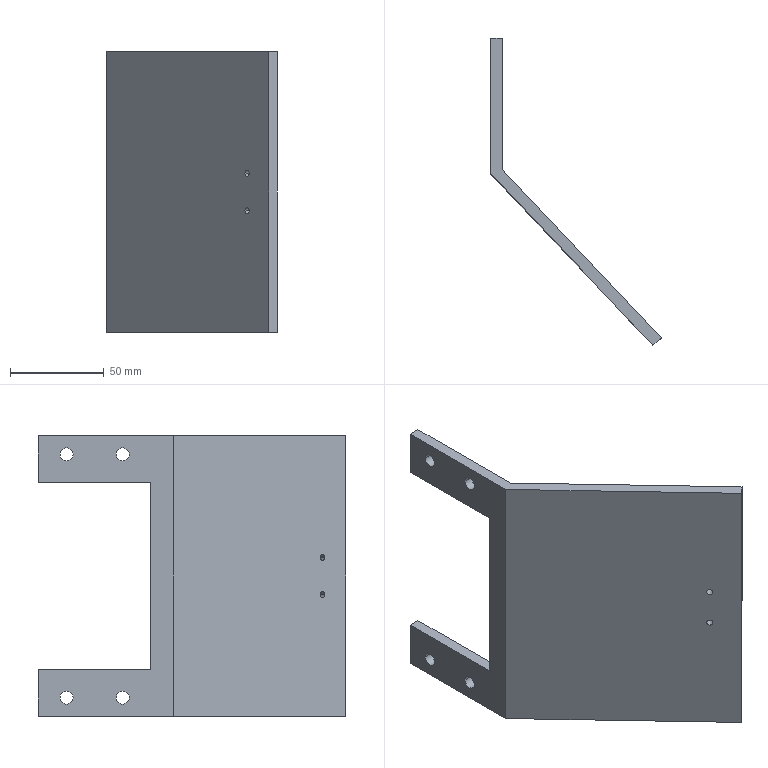Component | SolidWorks | ClampingMechanism-1_SupportPlate-1 | 1 solid | 24 faces | box 91 x 164.12 x 150 mm | volume 139535 mm3 | cylinder 12 | plane 12 | commonest cylinder face diameters 7 x8 3.3 x4
build123d program:
from build123d import *

# Parameters (mm, degrees)
BOSS_EXTRUDE1_DEPTH   = 75
SKETCH2_R             = 3.5
SKETCH2_W             = 120
SKETCH2_H             = 100
CUT_EXTRUDE1_DEPTH    = 10
M4_TAPPED_HOLE1_D     = 3.3
M4_TAPPED_HOLE1_DEPTH = 10.1
M4_TAPPED_HOLE1_TIP   = 0.9914


with BuildPart() as part:
    # Sketch1 → Boss-Extrude1 (new, symmetric)
    with BuildSketch(Plane.XY):
        Polygon((0, 0), (90, 85), (160, 85), (160, 91), (87.615, 91), (-4.12, 4.362), align=None)
    extrude(amount=BOSS_EXTRUDE1_DEPTH, both=True)

    # Sketch2 → Cut-Extrude1 (cut)
    with BuildSketch(Plane(origin=(0, 91, 0), x_dir=(1, 0, 0), z_dir=(0, 1, 0))):
        with Locations(Location((115, 65, 0), (0, 0, 180))):
            Circle(SKETCH2_R)
        with Locations(Location((145, 65, 0), (0, 0, 180))):
            Circle(SKETCH2_R)
        with Locations(Location((145, -65, 0), (0, 0, 180))):
            Circle(SKETCH2_R)
        with Locations(Location((115, -65, 0), (0, 0, 180))):
            Circle(SKETCH2_R)
        with Locations((160, 0)):
            Rectangle(SKETCH2_W, SKETCH2_H)
    extrude(amount=-CUT_EXTRUDE1_DEPTH, mode=Mode.SUBTRACT)

    # M4 Tapped Hole1
    with Locations(Plane(origin=(-4.12, 4.362, 0), x_dir=(0.727, 0.6866, 0), z_dir=(-0.6866, 0.727, 0))):
        with Locations((17, 10), (17, -10)):
            Hole(M4_TAPPED_HOLE1_D / 2, depth=M4_TAPPED_HOLE1_DEPTH)
            with Locations((0, 0, -(M4_TAPPED_HOLE1_DEPTH + M4_TAPPED_HOLE1_TIP / 2))):  # 118° drill point
                Cone(0, M4_TAPPED_HOLE1_D / 2, M4_TAPPED_HOLE1_TIP, mode=Mode.SUBTRACT)


solid = part.part

# Placed as in the assembly
solid = solid.moved(Location((-235, -250, -542.97), (0, 0, 90)))
STEP:
#1=COLOUR_RGB('',0.7922,0.8196,0.9333);
#2=FILL_AREA_STYLE_COLOUR('',#1);
#3=FILL_AREA_STYLE('',(#2));
#4=SURFACE_STYLE_FILL_AREA(#3);
#5=SURFACE_SIDE_STYLE('',(#4));
#6=SURFACE_STYLE_USAGE(.BOTH.,#5);
#7=PRESENTATION_STYLE_ASSIGNMENT((#6));
#8=CARTESIAN_POINT('',(-9.756,-9.309,-21.77));
#9=VERTEX_POINT('',#8);
#10=CARTESIAN_POINT('',(-9.667,-9.403,-21.77));
#11=VERTEX_POINT('',#10);
#12=CARTESIAN_POINT('',(-9.712,-9.356,-21.77));
#13=DIRECTION('',(-0.727,-0.6866,0.));
#14=DIRECTION('',(0.6866,-0.727,0.));
#15=AXIS2_PLACEMENT_3D('',#12,#13,#14);
#16=CIRCLE('',#15,0.06496);
#17=EDGE_CURVE('',#9,#11,#16,.T.);
#18=ORIENTED_EDGE('',*,*,#17,.F.);
#19=CARTESIAN_POINT('',(-9.928,-9.471,-21.77));
#20=VERTEX_POINT('',#19);
#21=CARTESIAN_POINT('',(-9.928,-9.471,-21.77));
#22=DIRECTION('',(-0.727,-0.6866,0.));
#23=VECTOR('',#22,39.37);
#24=LINE('',#21,#23);
#25=EDGE_CURVE('',#9,#20,#24,.T.);
#26=ORIENTED_EDGE('',*,*,#25,.T.);
#27=CARTESIAN_POINT('',(-9.839,-9.565,-21.77));
#28=VERTEX_POINT('',#27);
#29=CARTESIAN_POINT('',(-9.883,-9.518,-21.77));
#30=DIRECTION('',(-0.727,-0.6866,0.));
#31=DIRECTION('',(0.6866,-0.727,0.));
#32=AXIS2_PLACEMENT_3D('',#29,#30,#31);
#33=CIRCLE('',#32,0.06496);
#34=EDGE_CURVE('',#20,#28,#33,.T.);
#35=ORIENTED_EDGE('',*,*,#34,.T.);
#36=CARTESIAN_POINT('',(-9.839,-9.565,-21.77));
#37=DIRECTION('',(-0.727,-0.6866,0.));
#38=VECTOR('',#37,39.37);
#39=LINE('',#36,#38);
#40=EDGE_CURVE('',#11,#28,#39,.T.);
#41=ORIENTED_EDGE('',*,*,#40,.F.);
#42=EDGE_LOOP('',(#18,#26,#35,#41));
#43=FACE_OUTER_BOUND('',#42,.T.);
#44=CARTESIAN_POINT('',(-9.883,-9.518,-21.77));
#45=DIRECTION('',(-0.727,-0.6866,0.));
#46=DIRECTION('',(0.6866,-0.727,0.));
#47=AXIS2_PLACEMENT_3D('',#44,#45,#46);
#48=CYLINDRICAL_SURFACE('',#47,0.06496);
#49=ADVANCED_FACE('',(#43),#48,.F.);
#50=CARTESIAN_POINT('',(-9.756,-9.309,-20.983));
#51=VERTEX_POINT('',#50);
#52=CARTESIAN_POINT('',(-9.667,-9.403,-20.983));
#53=VERTEX_POINT('',#52);
#54=CARTESIAN_POINT('',(-9.712,-9.356,-20.983));
#55=DIRECTION('',(-0.727,-0.6866,0.));
#56=DIRECTION('',(0.6866,-0.727,0.));
#57=AXIS2_PLACEMENT_3D('',#54,#55,#56);
#58=CIRCLE('',#57,0.06496);
#59=EDGE_CURVE('',#51,#53,#58,.T.);
#60=ORIENTED_EDGE('',*,*,#59,.F.);
#61=CARTESIAN_POINT('',(-9.928,-9.471,-20.983));
#62=VERTEX_POINT('',#61);
#63=CARTESIAN_POINT('',(-9.928,-9.471,-20.983));
#64=DIRECTION('',(-0.727,-0.6866,0.));
#65=VECTOR('',#64,39.37);
#66=LINE('',#63,#65);
#67=EDGE_CURVE('',#51,#62,#66,.T.);
#68=ORIENTED_EDGE('',*,*,#67,.T.);
#69=CARTESIAN_POINT('',(-9.839,-9.565,-20.983));
#70=VERTEX_POINT('',#69);
#71=CARTESIAN_POINT('',(-9.883,-9.518,-20.983));
#72=DIRECTION('',(-0.727,-0.6866,0.));
#73=DIRECTION('',(0.6866,-0.727,0.));
#74=AXIS2_PLACEMENT_3D('',#71,#72,#73);
#75=CIRCLE('',#74,0.06496);
#76=EDGE_CURVE('',#62,#70,#75,.T.);
#77=ORIENTED_EDGE('',*,*,#76,.T.);
#78=CARTESIAN_POINT('',(-9.839,-9.565,-20.983));
#79=DIRECTION('',(-0.727,-0.6866,0.));
#80=VECTOR('',#79,39.37);
#81=LINE('',#78,#80);
#82=EDGE_CURVE('',#53,#70,#81,.T.);
#83=ORIENTED_EDGE('',*,*,#82,.F.);
#84=EDGE_LOOP('',(#60,#68,#77,#83));
#85=FACE_OUTER_BOUND('',#84,.T.);
#86=CARTESIAN_POINT('',(-9.883,-9.518,-20.983));
#87=DIRECTION('',(-0.727,-0.6866,0.));
#88=DIRECTION('',(0.6866,-0.727,0.));
#89=AXIS2_PLACEMENT_3D('',#86,#87,#88);
#90=CYLINDRICAL_SURFACE('',#89,0.06496);
#91=ADVANCED_FACE('',(#85),#90,.F.);
#92=CARTESIAN_POINT('',(-12.598,-5.177,-18.818));
#93=VERTEX_POINT('',#92);
#94=CARTESIAN_POINT('',(-12.598,-5.453,-18.818));
#95=VERTEX_POINT('',#94);
#96=CARTESIAN_POINT('',(-12.598,-5.315,-18.818));
#97=DIRECTION('',(-1.,0.,0.));
#98=DIRECTION('',(0.,-1.,0.));
#99=AXIS2_PLACEMENT_3D('',#96,#97,#98);
#100=CIRCLE('',#99,0.1378);
#101=EDGE_CURVE('',#93,#95,#100,.T.);
#102=ORIENTED_EDGE('',*,*,#101,.F.);
#103=CARTESIAN_POINT('',(-12.835,-5.177,-18.818));
#104=VERTEX_POINT('',#103);
#105=CARTESIAN_POINT('',(-12.441,-5.177,-18.818));
#106=DIRECTION('',(-1.,0.,0.));
#107=VECTOR('',#106,39.37);
#108=LINE('',#105,#107);
#109=EDGE_CURVE('',#93,#104,#108,.T.);
#110=ORIENTED_EDGE('',*,*,#109,.T.);
#111=CARTESIAN_POINT('',(-12.835,-5.453,-18.818));
#112=VERTEX_POINT('',#111);
#113=CARTESIAN_POINT('',(-12.835,-5.315,-18.818));
#114=DIRECTION('',(-1.,0.,0.));
#115=DIRECTION('',(0.,1.,0.));
#116=AXIS2_PLACEMENT_3D('',#113,#114,#115);
#117=CIRCLE('',#116,0.1378);
#118=EDGE_CURVE('',#104,#112,#117,.T.);
#119=ORIENTED_EDGE('',*,*,#118,.T.);
#120=CARTESIAN_POINT('',(-12.441,-5.453,-18.818));
#121=DIRECTION('',(-1.,0.,0.));
#122=VECTOR('',#121,39.37);
#123=LINE('',#120,#122);
#124=EDGE_CURVE('',#95,#112,#123,.T.);
#125=ORIENTED_EDGE('',*,*,#124,.F.);
#126=EDGE_LOOP('',(#102,#110,#119,#125));
#127=FACE_OUTER_BOUND('',#126,.T.);
#128=CARTESIAN_POINT('',(-12.441,-5.315,-18.818));
#129=DIRECTION('',(-1.,0.,0.));
#130=DIRECTION('',(0.,-1.,0.));
#131=AXIS2_PLACEMENT_3D('',#128,#129,#130);
#132=CYLINDRICAL_SURFACE('',#131,0.1378);
#133=ADVANCED_FACE('',(#127),#132,.F.);
#134=CARTESIAN_POINT('',(-12.598,-3.996,-18.818));
#135=VERTEX_POINT('',#134);
#136=CARTESIAN_POINT('',(-12.598,-4.272,-18.818));
#137=VERTEX_POINT('',#136);
#138=CARTESIAN_POINT('',(-12.598,-4.134,-18.818));
#139=DIRECTION('',(-1.,0.,0.));
#140=DIRECTION('',(0.,-1.,0.));
#141=AXIS2_PLACEMENT_3D('',#138,#139,#140);
#142=CIRCLE('',#141,0.1378);
#143=EDGE_CURVE('',#135,#137,#142,.T.);
#144=ORIENTED_EDGE('',*,*,#143,.F.);
#145=CARTESIAN_POINT('',(-12.835,-3.996,-18.818));
#146=VERTEX_POINT('',#145);
#147=CARTESIAN_POINT('',(-12.441,-3.996,-18.818));
#148=DIRECTION('',(-1.,0.,0.));
#149=VECTOR('',#148,39.37);
#150=LINE('',#147,#149);
#151=EDGE_CURVE('',#135,#146,#150,.T.);
#152=ORIENTED_EDGE('',*,*,#151,.T.);
#153=CARTESIAN_POINT('',(-12.835,-4.272,-18.818));
#154=VERTEX_POINT('',#153);
#155=CARTESIAN_POINT('',(-12.835,-4.134,-18.818));
#156=DIRECTION('',(-1.,0.,0.));
#157=DIRECTION('',(0.,1.,0.));
#158=AXIS2_PLACEMENT_3D('',#155,#156,#157);
#159=CIRCLE('',#158,0.1378);
#160=EDGE_CURVE('',#146,#154,#159,.T.);
#161=ORIENTED_EDGE('',*,*,#160,.T.);
#162=CARTESIAN_POINT('',(-12.441,-4.272,-18.818));
#163=DIRECTION('',(-1.,0.,0.));
#164=VECTOR('',#163,39.37);
#165=LINE('',#162,#164);
#166=EDGE_CURVE('',#137,#154,#165,.T.);
#167=ORIENTED_EDGE('',*,*,#166,.F.);
#168=EDGE_LOOP('',(#144,#152,#161,#167));
#169=FACE_OUTER_BOUND('',#168,.T.);
#170=CARTESIAN_POINT('',(-12.441,-4.134,-18.818));
#171=DIRECTION('',(-1.,0.,0.));
#172=DIRECTION('',(0.,-1.,0.));
#173=AXIS2_PLACEMENT_3D('',#170,#171,#172);
#174=CYLINDRICAL_SURFACE('',#173,0.1378);
#175=ADVANCED_FACE('',(#169),#174,.F.);
#176=CARTESIAN_POINT('',(-12.598,-3.996,-23.936));
#177=VERTEX_POINT('',#176);
#178=CARTESIAN_POINT('',(-12.598,-4.272,-23.936));
#179=VERTEX_POINT('',#178);
#180=CARTESIAN_POINT('',(-12.598,-4.134,-23.936));
#181=DIRECTION('',(-1.,0.,0.));
#182=DIRECTION('',(0.,-1.,0.));
#183=AXIS2_PLACEMENT_3D('',#180,#181,#182);
#184=CIRCLE('',#183,0.1378);
#185=EDGE_CURVE('',#177,#179,#184,.T.);
#186=ORIENTED_EDGE('',*,*,#185,.F.);
#187=CARTESIAN_POINT('',(-12.835,-3.996,-23.936));
#188=VERTEX_POINT('',#187);
#189=CARTESIAN_POINT('',(-12.441,-3.996,-23.936));
#190=DIRECTION('',(-1.,0.,0.));
#191=VECTOR('',#190,39.37);
#192=LINE('',#189,#191);
#193=EDGE_CURVE('',#177,#188,#192,.T.);
#194=ORIENTED_EDGE('',*,*,#193,.T.);
#195=CARTESIAN_POINT('',(-12.835,-4.272,-23.936));
#196=VERTEX_POINT('',#195);
#197=CARTESIAN_POINT('',(-12.835,-4.134,-23.936));
#198=DIRECTION('',(-1.,0.,0.));
#199=DIRECTION('',(0.,-1.,0.));
#200=AXIS2_PLACEMENT_3D('',#197,#198,#199);
#201=CIRCLE('',#200,0.1378);
#202=EDGE_CURVE('',#188,#196,#201,.T.);
#203=ORIENTED_EDGE('',*,*,#202,.T.);
#204=CARTESIAN_POINT('',(-12.441,-4.272,-23.936));
#205=DIRECTION('',(-1.,0.,0.));
#206=VECTOR('',#205,39.37);
#207=LINE('',#204,#206);
#208=EDGE_CURVE('',#179,#196,#207,.T.);
#209=ORIENTED_EDGE('',*,*,#208,.F.);
#210=EDGE_LOOP('',(#186,#194,#203,#209));
#211=FACE_OUTER_BOUND('',#210,.T.);
#212=CARTESIAN_POINT('',(-12.441,-4.134,-23.936));
#213=DIRECTION('',(-1.,0.,0.));
#214=DIRECTION('',(0.,-1.,0.));
#215=AXIS2_PLACEMENT_3D('',#212,#213,#214);
#216=CYLINDRICAL_SURFACE('',#215,0.1378);
#217=ADVANCED_FACE('',(#211),#216,.F.);
#218=CARTESIAN_POINT('',(-12.598,-5.177,-23.936));
#219=VERTEX_POINT('',#218);
#220=CARTESIAN_POINT('',(-12.598,-5.453,-23.936));
#221=VERTEX_POINT('',#220);
#222=CARTESIAN_POINT('',(-12.598,-5.315,-23.936));
#223=DIRECTION('',(-1.,0.,0.));
#224=DIRECTION('',(0.,-1.,0.));
#225=AXIS2_PLACEMENT_3D('',#222,#223,#224);
#226=CIRCLE('',#225,0.1378);
#227=EDGE_CURVE('',#219,#221,#226,.T.);
#228=ORIENTED_EDGE('',*,*,#227,.F.);
#229=CARTESIAN_POINT('',(-12.835,-5.177,-23.936));
#230=VERTEX_POINT('',#229);
#231=CARTESIAN_POINT('',(-12.441,-5.177,-23.936));
#232=DIRECTION('',(-1.,0.,0.));
#233=VECTOR('',#232,39.37);
#234=LINE('',#231,#233);
#235=EDGE_CURVE('',#219,#230,#234,.T.);
#236=ORIENTED_EDGE('',*,*,#235,.T.);
#237=CARTESIAN_POINT('',(-12.835,-5.453,-23.936));
#238=VERTEX_POINT('',#237);
#239=CARTESIAN_POINT('',(-12.835,-5.315,-23.936));
#240=DIRECTION('',(-1.,0.,0.));
#241=DIRECTION('',(0.,-1.,0.));
#242=AXIS2_PLACEMENT_3D('',#239,#240,#241);
#243=CIRCLE('',#242,0.1378);
#244=EDGE_CURVE('',#230,#238,#243,.T.);
#245=ORIENTED_EDGE('',*,*,#244,.T.);
#246=CARTESIAN_POINT('',(-12.441,-5.453,-23.936));
#247=DIRECTION('',(-1.,0.,0.));
#248=VECTOR('',#247,39.37);
#249=LINE('',#246,#248);
#250=EDGE_CURVE('',#221,#238,#249,.T.);
#251=ORIENTED_EDGE('',*,*,#250,.F.);
#252=EDGE_LOOP('',(#228,#236,#245,#251));
#253=FACE_OUTER_BOUND('',#252,.T.);
#254=CARTESIAN_POINT('',(-12.441,-5.315,-23.936));
#255=DIRECTION('',(-1.,0.,0.));
#256=DIRECTION('',(0.,-1.,0.));
#257=AXIS2_PLACEMENT_3D('',#254,#255,#256);
#258=CYLINDRICAL_SURFACE('',#257,0.1378);
#259=ADVANCED_FACE('',(#253),#258,.F.);
#260=CARTESIAN_POINT('',(-12.598,-3.543,-18.424));
#261=VERTEX_POINT('',#260);
#262=CARTESIAN_POINT('',(-12.598,-3.543,-19.408));
#263=VERTEX_POINT('',#262);
#264=CARTESIAN_POINT('',(-12.598,-3.543,-18.424));
#265=DIRECTION('',(-0.,0.,-1.));
#266=VECTOR('',#265,39.37);
#267=LINE('',#264,#266);
#268=EDGE_CURVE('',#261,#263,#267,.T.);
#269=ORIENTED_EDGE('',*,*,#268,.T.);
#270=CARTESIAN_POINT('',(-12.835,-3.543,-19.408));
#271=VERTEX_POINT('',#270);
#272=CARTESIAN_POINT('',(-12.835,-3.543,-19.408));
#273=DIRECTION('',(-1.,-0.,0.));
#274=VECTOR('',#273,39.37);
#275=LINE('',#272,#274);
#276=EDGE_CURVE('',#263,#271,#275,.T.);
#277=ORIENTED_EDGE('',*,*,#276,.T.);
#278=CARTESIAN_POINT('',(-12.835,-3.543,-18.424));
#279=VERTEX_POINT('',#278);
#280=CARTESIAN_POINT('',(-12.835,-3.543,-18.424));
#281=DIRECTION('',(-0.,0.,-1.));
#282=VECTOR('',#281,39.37);
#283=LINE('',#280,#282);
#284=EDGE_CURVE('',#279,#271,#283,.T.);
#285=ORIENTED_EDGE('',*,*,#284,.F.);
#286=CARTESIAN_POINT('',(-12.835,-3.543,-18.424));
#287=DIRECTION('',(-1.,-0.,0.));
#288=VECTOR('',#287,39.37);
#289=LINE('',#286,#288);
#290=EDGE_CURVE('',#261,#279,#289,.T.);
#291=ORIENTED_EDGE('',*,*,#290,.F.);
#292=EDGE_LOOP('',(#269,#277,#285,#291));
#293=FACE_OUTER_BOUND('',#292,.T.);
#294=CARTESIAN_POINT('',(-12.835,-3.543,-18.424));
#295=DIRECTION('',(0.,-1.,-0.));
#296=DIRECTION('',(0.,-0.,1.));
#297=AXIS2_PLACEMENT_3D('',#294,#295,#296);
#298=PLANE('',#297);
#299=ADVANCED_FACE('',(#293),#298,.F.);
#300=CARTESIAN_POINT('',(-9.424,-10.005,-24.33));
#301=VERTEX_POINT('',#300);
#302=CARTESIAN_POINT('',(-9.252,-9.843,-24.33));
#303=VERTEX_POINT('',#302);
#304=CARTESIAN_POINT('',(-9.424,-10.005,-24.33));
#305=DIRECTION('',(0.727,0.6866,-0.));
#306=VECTOR('',#305,39.37);
#307=LINE('',#304,#306);
#308=EDGE_CURVE('',#301,#303,#307,.T.);
#309=ORIENTED_EDGE('',*,*,#308,.T.);
#310=CARTESIAN_POINT('',(-9.252,-9.843,-18.424));
#311=VERTEX_POINT('',#310);
#312=CARTESIAN_POINT('',(-9.252,-9.843,-18.424));
#313=DIRECTION('',(-0.,0.,-1.));
#314=VECTOR('',#313,39.37);
#315=LINE('',#312,#314);
#316=EDGE_CURVE('',#311,#303,#315,.T.);
#317=ORIENTED_EDGE('',*,*,#316,.F.);
#318=CARTESIAN_POINT('',(-9.424,-10.005,-18.424));
#319=VERTEX_POINT('',#318);
#320=CARTESIAN_POINT('',(-9.424,-10.005,-18.424));
#321=DIRECTION('',(0.727,0.6866,-0.));
#322=VECTOR('',#321,39.37);
#323=LINE('',#320,#322);
#324=EDGE_CURVE('',#319,#311,#323,.T.);
#325=ORIENTED_EDGE('',*,*,#324,.F.);
#326=CARTESIAN_POINT('',(-9.424,-10.005,-18.424));
#327=DIRECTION('',(-0.,0.,-1.));
#328=VECTOR('',#327,39.37);
#329=LINE('',#326,#328);
#330=EDGE_CURVE('',#319,#301,#329,.T.);
#331=ORIENTED_EDGE('',*,*,#330,.T.);
#332=EDGE_LOOP('',(#309,#317,#325,#331));
#333=FACE_OUTER_BOUND('',#332,.T.);
#334=CARTESIAN_POINT('',(-9.424,-10.005,-18.424));
#335=DIRECTION('',(-0.6866,0.727,0.));
#336=DIRECTION('',(-0.727,-0.6866,0.));
#337=AXIS2_PLACEMENT_3D('',#334,#335,#336);
#338=PLANE('',#337);
#339=ADVANCED_FACE('',(#333),#338,.F.);
#340=CARTESIAN_POINT('',(-9.712,-9.356,-21.77));
#341=DIRECTION('',(-0.727,-0.6866,0.));
#342=DIRECTION('',(0.6866,-0.727,0.));
#343=AXIS2_PLACEMENT_3D('',#340,#341,#342);
#344=CIRCLE('',#343,0.06496);
#345=EDGE_CURVE('',#11,#9,#344,.T.);
#346=ORIENTED_EDGE('',*,*,#345,.T.);
#347=ORIENTED_EDGE('',*,*,#17,.T.);
#348=EDGE_LOOP('',(#346,#347));
#349=FACE_BOUND('',#348,.T.);
#350=CARTESIAN_POINT('',(-9.712,-9.356,-20.983));
#351=DIRECTION('',(-0.727,-0.6866,0.));
#352=DIRECTION('',(0.6866,-0.727,0.));
#353=AXIS2_PLACEMENT_3D('',#350,#351,#352);
#354=CIRCLE('',#353,0.06496);
#355=EDGE_CURVE('',#53,#51,#354,.T.);
#356=ORIENTED_EDGE('',*,*,#355,.T.);
#357=ORIENTED_EDGE('',*,*,#59,.T.);
#358=EDGE_LOOP('',(#356,#357));
#359=FACE_BOUND('',#358,.T.);
#360=CARTESIAN_POINT('',(-12.598,-6.299,-24.33));
#361=VERTEX_POINT('',#360);
#362=CARTESIAN_POINT('',(-9.252,-9.843,-24.33));
#363=DIRECTION('',(-0.6866,0.727,0.));
#364=VECTOR('',#363,39.37);
#365=LINE('',#362,#364);
#366=EDGE_CURVE('',#303,#361,#365,.T.);
#367=ORIENTED_EDGE('',*,*,#366,.T.);
#368=CARTESIAN_POINT('',(-12.598,-6.299,-18.424));
#369=VERTEX_POINT('',#368);
#370=CARTESIAN_POINT('',(-12.598,-6.299,-18.424));
#371=DIRECTION('',(-0.,0.,-1.));
#372=VECTOR('',#371,39.37);
#373=LINE('',#370,#372);
#374=EDGE_CURVE('',#369,#361,#373,.T.);
#375=ORIENTED_EDGE('',*,*,#374,.F.);
#376=CARTESIAN_POINT('',(-9.252,-9.843,-18.424));
#377=DIRECTION('',(-0.6866,0.727,0.));
#378=VECTOR('',#377,39.37);
#379=LINE('',#376,#378);
#380=EDGE_CURVE('',#311,#369,#379,.T.);
#381=ORIENTED_EDGE('',*,*,#380,.F.);
#382=ORIENTED_EDGE('',*,*,#316,.T.);
#383=EDGE_LOOP('',(#367,#375,#381,#382));
#384=FACE_OUTER_BOUND('',#383,.T.);
#385=CARTESIAN_POINT('',(-9.252,-9.843,-18.424));
#386=DIRECTION('',(-0.727,-0.6866,0.));
#387=DIRECTION('',(0.6866,-0.727,-0.));
#388=AXIS2_PLACEMENT_3D('',#385,#386,#387);
#389=PLANE('',#388);
#390=ADVANCED_FACE('',(#349,#359,#384),#389,.F.);
#391=CARTESIAN_POINT('',(-12.598,-5.315,-18.818));
#392=DIRECTION('',(-1.,0.,0.));
#393=DIRECTION('',(0.,-1.,0.));
#394=AXIS2_PLACEMENT_3D('',#391,#392,#393);
#395=CIRCLE('',#394,0.1378);
#396=EDGE_CURVE('',#95,#93,#395,.T.);
#397=ORIENTED_EDGE('',*,*,#396,.T.);
#398=ORIENTED_EDGE('',*,*,#101,.T.);
#399=EDGE_LOOP('',(#397,#398));
#400=FACE_BOUND('',#399,.T.);
#401=CARTESIAN_POINT('',(-12.598,-4.134,-18.818));
#402=DIRECTION('',(-1.,0.,0.));
#403=DIRECTION('',(0.,-1.,0.));
#404=AXIS2_PLACEMENT_3D('',#401,#402,#403);
#405=CIRCLE('',#404,0.1378);
#406=EDGE_CURVE('',#137,#135,#405,.T.);
#407=ORIENTED_EDGE('',*,*,#406,.T.);
#408=ORIENTED_EDGE('',*,*,#143,.T.);
#409=EDGE_LOOP('',(#407,#408));
#410=FACE_BOUND('',#409,.T.);
#411=CARTESIAN_POINT('',(-12.598,-4.134,-23.936));
#412=DIRECTION('',(-1.,0.,0.));
#413=DIRECTION('',(0.,-1.,0.));
#414=AXIS2_PLACEMENT_3D('',#411,#412,#413);
#415=CIRCLE('',#414,0.1378);
#416=EDGE_CURVE('',#179,#177,#415,.T.);
#417=ORIENTED_EDGE('',*,*,#416,.T.);
#418=ORIENTED_EDGE('',*,*,#185,.T.);
#419=EDGE_LOOP('',(#417,#418));
#420=FACE_BOUND('',#419,.T.);
#421=CARTESIAN_POINT('',(-12.598,-5.315,-23.936));
#422=DIRECTION('',(-1.,0.,0.));
#423=DIRECTION('',(0.,-1.,0.));
#424=AXIS2_PLACEMENT_3D('',#421,#422,#423);
#425=CIRCLE('',#424,0.1378);
#426=EDGE_CURVE('',#221,#219,#425,.T.);
#427=ORIENTED_EDGE('',*,*,#426,.T.);
#428=ORIENTED_EDGE('',*,*,#227,.T.);
#429=EDGE_LOOP('',(#427,#428));
#430=FACE_BOUND('',#429,.T.);
#431=CARTESIAN_POINT('',(-12.598,-5.906,-23.345));
#432=VERTEX_POINT('',#431);
#433=CARTESIAN_POINT('',(-12.598,-5.906,-19.408));
#434=VERTEX_POINT('',#433);
#435=CARTESIAN_POINT('',(-12.598,-5.906,-18.424));
#436=DIRECTION('',(0.,-0.,1.));
#437=VECTOR('',#436,39.37);
#438=LINE('',#435,#437);
#439=EDGE_CURVE('',#432,#434,#438,.T.);
#440=ORIENTED_EDGE('',*,*,#439,.T.);
#441=CARTESIAN_POINT('',(-12.598,-6.299,-19.408));
#442=DIRECTION('',(0.,1.,0.));
#443=VECTOR('',#442,39.37);
#444=LINE('',#441,#443);
#445=EDGE_CURVE('',#434,#263,#444,.T.);
#446=ORIENTED_EDGE('',*,*,#445,.T.);
#447=ORIENTED_EDGE('',*,*,#268,.F.);
#448=CARTESIAN_POINT('',(-12.598,-6.299,-18.424));
#449=DIRECTION('',(0.,1.,0.));
#450=VECTOR('',#449,39.37);
#451=LINE('',#448,#450);
#452=EDGE_CURVE('',#369,#261,#451,.T.);
#453=ORIENTED_EDGE('',*,*,#452,.F.);
#454=ORIENTED_EDGE('',*,*,#374,.T.);
#455=CARTESIAN_POINT('',(-12.598,-3.543,-24.33));
#456=VERTEX_POINT('',#455);
#457=CARTESIAN_POINT('',(-12.598,-6.299,-24.33));
#458=DIRECTION('',(0.,1.,0.));
#459=VECTOR('',#458,39.37);
#460=LINE('',#457,#459);
#461=EDGE_CURVE('',#361,#456,#460,.T.);
#462=ORIENTED_EDGE('',*,*,#461,.T.);
#463=CARTESIAN_POINT('',(-12.598,-3.543,-23.345));
#464=VERTEX_POINT('',#463);
#465=CARTESIAN_POINT('',(-12.598,-3.543,-18.424));
#466=DIRECTION('',(-0.,0.,-1.));
#467=VECTOR('',#466,39.37);
#468=LINE('',#465,#467);
#469=EDGE_CURVE('',#464,#456,#468,.T.);
#470=ORIENTED_EDGE('',*,*,#469,.F.);
#471=CARTESIAN_POINT('',(-12.598,-6.299,-23.345));
#472=DIRECTION('',(-0.,-1.,-0.));
#473=VECTOR('',#472,39.37);
#474=LINE('',#471,#473);
#475=EDGE_CURVE('',#464,#432,#474,.T.);
#476=ORIENTED_EDGE('',*,*,#475,.T.);
#477=EDGE_LOOP('',(#440,#446,#447,#453,#454,#462,#470,#476));
#478=FACE_OUTER_BOUND('',#477,.T.);
#479=CARTESIAN_POINT('',(-12.598,-6.299,-18.424));
#480=DIRECTION('',(-1.,0.,0.));
#481=DIRECTION('',(-0.,-1.,-0.));
#482=AXIS2_PLACEMENT_3D('',#479,#480,#481);
#483=PLANE('',#482);
#484=ADVANCED_FACE('',(#400,#410,#420,#430,#478),#483,.F.);
#485=CARTESIAN_POINT('',(-12.835,-3.543,-23.345));
#486=VERTEX_POINT('',#485);
#487=CARTESIAN_POINT('',(-12.835,-3.543,-24.33));
#488=VERTEX_POINT('',#487);
#489=CARTESIAN_POINT('',(-12.835,-3.543,-18.424));
#490=DIRECTION('',(-0.,0.,-1.));
#491=VECTOR('',#490,39.37);
#492=LINE('',#489,#491);
#493=EDGE_CURVE('',#486,#488,#492,.T.);
#494=ORIENTED_EDGE('',*,*,#493,.F.);
#495=CARTESIAN_POINT('',(-12.835,-3.543,-23.345));
#496=DIRECTION('',(1.,0.,-0.));
#497=VECTOR('',#496,39.37);
#498=LINE('',#495,#497);
#499=EDGE_CURVE('',#486,#464,#498,.T.);
#500=ORIENTED_EDGE('',*,*,#499,.T.);
#501=ORIENTED_EDGE('',*,*,#469,.T.);
#502=CARTESIAN_POINT('',(-12.835,-3.543,-24.33));
#503=DIRECTION('',(-1.,-0.,0.));
#504=VECTOR('',#503,39.37);
#505=LINE('',#502,#504);
#506=EDGE_CURVE('',#456,#488,#505,.T.);
#507=ORIENTED_EDGE('',*,*,#506,.T.);
#508=EDGE_LOOP('',(#494,#500,#501,#507));
#509=FACE_OUTER_BOUND('',#508,.T.);
#510=CARTESIAN_POINT('',(-12.835,-3.543,-18.424));
#511=DIRECTION('',(0.,-1.,-0.));
#512=DIRECTION('',(0.,-0.,1.));
#513=AXIS2_PLACEMENT_3D('',#510,#511,#512);
#514=PLANE('',#513);
#515=ADVANCED_FACE('',(#509),#514,.F.);
#516=CARTESIAN_POINT('',(-12.835,-5.315,-18.818));
#517=DIRECTION('',(-1.,0.,0.));
#518=DIRECTION('',(0.,1.,0.));
#519=AXIS2_PLACEMENT_3D('',#516,#517,#518);
#520=CIRCLE('',#519,0.1378);
#521=EDGE_CURVE('',#112,#104,#520,.T.);
#522=ORIENTED_EDGE('',*,*,#521,.F.);
#523=ORIENTED_EDGE('',*,*,#118,.F.);
#524=EDGE_LOOP('',(#522,#523));
#525=FACE_BOUND('',#524,.T.);
#526=CARTESIAN_POINT('',(-12.835,-4.134,-18.818));
#527=DIRECTION('',(-1.,0.,0.));
#528=DIRECTION('',(0.,1.,0.));
#529=AXIS2_PLACEMENT_3D('',#526,#527,#528);
#530=CIRCLE('',#529,0.1378);
#531=EDGE_CURVE('',#154,#146,#530,.T.);
#532=ORIENTED_EDGE('',*,*,#531,.F.);
#533=ORIENTED_EDGE('',*,*,#160,.F.);
#534=EDGE_LOOP('',(#532,#533));
#535=FACE_BOUND('',#534,.T.);
#536=CARTESIAN_POINT('',(-12.835,-4.134,-23.936));
#537=DIRECTION('',(-1.,0.,0.));
#538=DIRECTION('',(0.,-1.,0.));
#539=AXIS2_PLACEMENT_3D('',#536,#537,#538);
#540=CIRCLE('',#539,0.1378);
#541=EDGE_CURVE('',#196,#188,#540,.T.);
#542=ORIENTED_EDGE('',*,*,#541,.F.);
#543=ORIENTED_EDGE('',*,*,#202,.F.);
#544=EDGE_LOOP('',(#542,#543));
#545=FACE_BOUND('',#544,.T.);
#546=CARTESIAN_POINT('',(-12.835,-5.315,-23.936));
#547=DIRECTION('',(-1.,0.,0.));
#548=DIRECTION('',(0.,-1.,0.));
#549=AXIS2_PLACEMENT_3D('',#546,#547,#548);
#550=CIRCLE('',#549,0.1378);
#551=EDGE_CURVE('',#238,#230,#550,.T.);
#552=ORIENTED_EDGE('',*,*,#551,.F.);
#553=ORIENTED_EDGE('',*,*,#244,.F.);
#554=EDGE_LOOP('',(#552,#553));
#555=FACE_BOUND('',#554,.T.);
#556=ORIENTED_EDGE('',*,*,#284,.T.);
#557=CARTESIAN_POINT('',(-12.835,-5.906,-19.408));
#558=VERTEX_POINT('',#557);
#559=CARTESIAN_POINT('',(-12.835,-5.906,-19.408));
#560=DIRECTION('',(0.,1.,0.));
#561=VECTOR('',#560,39.37);
#562=LINE('',#559,#561);
#563=EDGE_CURVE('',#558,#271,#562,.T.);
#564=ORIENTED_EDGE('',*,*,#563,.F.);
#565=CARTESIAN_POINT('',(-12.835,-5.906,-23.345));
#566=VERTEX_POINT('',#565);
#567=CARTESIAN_POINT('',(-12.835,-5.906,-23.345));
#568=DIRECTION('',(0.,-0.,1.));
#569=VECTOR('',#568,39.37);
#570=LINE('',#567,#569);
#571=EDGE_CURVE('',#566,#558,#570,.T.);
#572=ORIENTED_EDGE('',*,*,#571,.F.);
#573=CARTESIAN_POINT('',(-12.835,-6.393,-23.345));
#574=DIRECTION('',(-0.,1.,0.));
#575=VECTOR('',#574,39.37);
#576=LINE('',#573,#575);
#577=EDGE_CURVE('',#566,#486,#576,.T.);
#578=ORIENTED_EDGE('',*,*,#577,.T.);
#579=ORIENTED_EDGE('',*,*,#493,.T.);
#580=CARTESIAN_POINT('',(-12.835,-6.393,-24.33));
#581=VERTEX_POINT('',#580);
#582=CARTESIAN_POINT('',(-12.835,-6.393,-24.33));
#583=DIRECTION('',(0.,-1.,-0.));
#584=VECTOR('',#583,39.37);
#585=LINE('',#582,#584);
#586=EDGE_CURVE('',#488,#581,#585,.T.);
#587=ORIENTED_EDGE('',*,*,#586,.T.);
#588=CARTESIAN_POINT('',(-12.835,-6.393,-18.424));
#589=VERTEX_POINT('',#588);
#590=CARTESIAN_POINT('',(-12.835,-6.393,-18.424));
#591=DIRECTION('',(-0.,0.,-1.));
#592=VECTOR('',#591,39.37);
#593=LINE('',#590,#592);
#594=EDGE_CURVE('',#589,#581,#593,.T.);
#595=ORIENTED_EDGE('',*,*,#594,.F.);
#596=CARTESIAN_POINT('',(-12.835,-6.393,-18.424));
#597=DIRECTION('',(0.,-1.,-0.));
#598=VECTOR('',#597,39.37);
#599=LINE('',#596,#598);
#600=EDGE_CURVE('',#279,#589,#599,.T.);
#601=ORIENTED_EDGE('',*,*,#600,.F.);
#602=EDGE_LOOP('',(#556,#564,#572,#578,#579,#587,#595,#601));
#603=FACE_OUTER_BOUND('',#602,.T.);
#604=CARTESIAN_POINT('',(-12.835,-6.393,-18.424));
#605=DIRECTION('',(1.,0.,-0.));
#606=DIRECTION('',(-0.,0.,-1.));
#607=AXIS2_PLACEMENT_3D('',#604,#605,#606);
#608=PLANE('',#607);
#609=ADVANCED_FACE('',(#525,#535,#545,#555,#603),#608,.F.);
#610=CARTESIAN_POINT('',(-9.883,-9.518,-21.77));
#611=DIRECTION('',(-0.727,-0.6866,0.));
#612=DIRECTION('',(0.6866,-0.727,0.));
#613=AXIS2_PLACEMENT_3D('',#610,#611,#612);
#614=CIRCLE('',#613,0.06496);
#615=EDGE_CURVE('',#28,#20,#614,.T.);
#616=ORIENTED_EDGE('',*,*,#615,.F.);
#617=ORIENTED_EDGE('',*,*,#34,.F.);
#618=EDGE_LOOP('',(#616,#617));
#619=FACE_BOUND('',#618,.T.);
#620=CARTESIAN_POINT('',(-9.883,-9.518,-20.983));
#621=DIRECTION('',(-0.727,-0.6866,0.));
#622=DIRECTION('',(0.6866,-0.727,0.));
#623=AXIS2_PLACEMENT_3D('',#620,#621,#622);
#624=CIRCLE('',#623,0.06496);
#625=EDGE_CURVE('',#70,#62,#624,.T.);
#626=ORIENTED_EDGE('',*,*,#625,.F.);
#627=ORIENTED_EDGE('',*,*,#76,.F.);
#628=EDGE_LOOP('',(#626,#627));
#629=FACE_BOUND('',#628,.T.);
#630=CARTESIAN_POINT('',(-9.424,-10.005,-24.33));
#631=DIRECTION('',(0.6866,-0.727,-0.));
#632=VECTOR('',#631,39.37);
#633=LINE('',#630,#632);
#634=EDGE_CURVE('',#581,#301,#633,.T.);
#635=ORIENTED_EDGE('',*,*,#634,.T.);
#636=ORIENTED_EDGE('',*,*,#330,.F.);
#637=CARTESIAN_POINT('',(-9.424,-10.005,-18.424));
#638=DIRECTION('',(0.6866,-0.727,-0.));
#639=VECTOR('',#638,39.37);
#640=LINE('',#637,#639);
#641=EDGE_CURVE('',#589,#319,#640,.T.);
#642=ORIENTED_EDGE('',*,*,#641,.F.);
#643=ORIENTED_EDGE('',*,*,#594,.T.);
#644=EDGE_LOOP('',(#635,#636,#642,#643));
#645=FACE_OUTER_BOUND('',#644,.T.);
#646=CARTESIAN_POINT('',(-9.424,-10.005,-18.424));
#647=DIRECTION('',(0.727,0.6866,-0.));
#648=DIRECTION('',(-0.6866,0.727,0.));
#649=AXIS2_PLACEMENT_3D('',#646,#647,#648);
#650=PLANE('',#649);
#651=ADVANCED_FACE('',(#619,#629,#645),#650,.F.);
#652=ORIENTED_EDGE('',*,*,#324,.T.);
#653=ORIENTED_EDGE('',*,*,#380,.T.);
#654=ORIENTED_EDGE('',*,*,#452,.T.);
#655=ORIENTED_EDGE('',*,*,#290,.T.);
#656=ORIENTED_EDGE('',*,*,#600,.T.);
#657=ORIENTED_EDGE('',*,*,#641,.T.);
#658=EDGE_LOOP('',(#652,#653,#654,#655,#656,#657));
#659=FACE_OUTER_BOUND('',#658,.T.);
#660=CARTESIAN_POINT('',(-9.252,-9.843,-18.424));
#661=DIRECTION('',(0.,-0.,1.));
#662=DIRECTION('',(-0.,1.,0.));
#663=AXIS2_PLACEMENT_3D('',#660,#661,#662);
#664=PLANE('',#663);
#665=ADVANCED_FACE('',(#659),#664,.T.);
#666=ORIENTED_EDGE('',*,*,#308,.F.);
#667=ORIENTED_EDGE('',*,*,#634,.F.);
#668=ORIENTED_EDGE('',*,*,#586,.F.);
#669=ORIENTED_EDGE('',*,*,#506,.F.);
#670=ORIENTED_EDGE('',*,*,#461,.F.);
#671=ORIENTED_EDGE('',*,*,#366,.F.);
#672=EDGE_LOOP('',(#666,#667,#668,#669,#670,#671));
#673=FACE_OUTER_BOUND('',#672,.T.);
#674=CARTESIAN_POINT('',(-9.252,-9.843,-24.33));
#675=DIRECTION('',(0.,-0.,1.));
#676=DIRECTION('',(-0.,1.,0.));
#677=AXIS2_PLACEMENT_3D('',#674,#675,#676);
#678=PLANE('',#677);
#679=ADVANCED_FACE('',(#673),#678,.F.);
#680=CARTESIAN_POINT('',(-12.441,-5.906,-19.408));
#681=DIRECTION('',(-1.,0.,0.));
#682=VECTOR('',#681,39.37);
#683=LINE('',#680,#682);
#684=EDGE_CURVE('',#434,#558,#683,.T.);
#685=ORIENTED_EDGE('',*,*,#684,.T.);
#686=ORIENTED_EDGE('',*,*,#563,.T.);
#687=ORIENTED_EDGE('',*,*,#276,.F.);
#688=ORIENTED_EDGE('',*,*,#445,.F.);
#689=EDGE_LOOP('',(#685,#686,#687,#688));
#690=FACE_OUTER_BOUND('',#689,.T.);
#691=CARTESIAN_POINT('',(-12.441,-5.906,-19.408));
#692=DIRECTION('',(0.,-0.,1.));
#693=DIRECTION('',(-0.,1.,0.));
#694=AXIS2_PLACEMENT_3D('',#691,#692,#693);
#695=PLANE('',#694);
#696=ADVANCED_FACE('',(#690),#695,.F.);
#697=CARTESIAN_POINT('',(-12.441,-5.906,-23.345));
#698=DIRECTION('',(-1.,0.,0.));
#699=VECTOR('',#698,39.37);
#700=LINE('',#697,#699);
#701=EDGE_CURVE('',#432,#566,#700,.T.);
#702=ORIENTED_EDGE('',*,*,#701,.T.);
#703=ORIENTED_EDGE('',*,*,#571,.T.);
#704=ORIENTED_EDGE('',*,*,#684,.F.);
#705=ORIENTED_EDGE('',*,*,#439,.F.);
#706=EDGE_LOOP('',(#702,#703,#704,#705));
#707=FACE_OUTER_BOUND('',#706,.T.);
#708=CARTESIAN_POINT('',(-12.441,-5.906,-23.345));
#709=DIRECTION('',(-0.,-1.,-0.));
#710=DIRECTION('',(1.,-0.,-0.));
#711=AXIS2_PLACEMENT_3D('',#708,#709,#710);
#712=PLANE('',#711);
#713=ADVANCED_FACE('',(#707),#712,.F.);
#714=ORIENTED_EDGE('',*,*,#499,.F.);
#715=ORIENTED_EDGE('',*,*,#577,.F.);
#716=ORIENTED_EDGE('',*,*,#701,.F.);
#717=ORIENTED_EDGE('',*,*,#475,.F.);
#718=EDGE_LOOP('',(#714,#715,#716,#717));
#719=FACE_OUTER_BOUND('',#718,.T.);
#720=CARTESIAN_POINT('',(-12.441,-5.906,-23.345));
#721=DIRECTION('',(-0.,0.,-1.));
#722=DIRECTION('',(0.,-1.,-0.));
#723=AXIS2_PLACEMENT_3D('',#720,#721,#722);
#724=PLANE('',#723);
#725=ADVANCED_FACE('',(#719),#724,.F.);
#726=ORIENTED_EDGE('',*,*,#235,.F.);
#727=ORIENTED_EDGE('',*,*,#426,.F.);
#728=ORIENTED_EDGE('',*,*,#250,.T.);
#729=ORIENTED_EDGE('',*,*,#551,.T.);
#730=EDGE_LOOP('',(#726,#727,#728,#729));
#731=FACE_OUTER_BOUND('',#730,.T.);
#732=CARTESIAN_POINT('',(-12.441,-5.315,-23.936));
#733=DIRECTION('',(-1.,0.,0.));
#734=DIRECTION('',(0.,-1.,0.));
#735=AXIS2_PLACEMENT_3D('',#732,#733,#734);
#736=CYLINDRICAL_SURFACE('',#735,0.1378);
#737=ADVANCED_FACE('',(#731),#736,.F.);
#738=ORIENTED_EDGE('',*,*,#193,.F.);
#739=ORIENTED_EDGE('',*,*,#416,.F.);
#740=ORIENTED_EDGE('',*,*,#208,.T.);
#741=ORIENTED_EDGE('',*,*,#541,.T.);
#742=EDGE_LOOP('',(#738,#739,#740,#741));
#743=FACE_OUTER_BOUND('',#742,.T.);
#744=CARTESIAN_POINT('',(-12.441,-4.134,-23.936));
#745=DIRECTION('',(-1.,0.,0.));
#746=DIRECTION('',(0.,-1.,0.));
#747=AXIS2_PLACEMENT_3D('',#744,#745,#746);
#748=CYLINDRICAL_SURFACE('',#747,0.1378);
#749=ADVANCED_FACE('',(#743),#748,.F.);
#750=ORIENTED_EDGE('',*,*,#151,.F.);
#751=ORIENTED_EDGE('',*,*,#406,.F.);
#752=ORIENTED_EDGE('',*,*,#166,.T.);
#753=ORIENTED_EDGE('',*,*,#531,.T.);
#754=EDGE_LOOP('',(#750,#751,#752,#753));
#755=FACE_OUTER_BOUND('',#754,.T.);
#756=CARTESIAN_POINT('',(-12.441,-4.134,-18.818));
#757=DIRECTION('',(-1.,0.,0.));
#758=DIRECTION('',(0.,-1.,0.));
#759=AXIS2_PLACEMENT_3D('',#756,#757,#758);
#760=CYLINDRICAL_SURFACE('',#759,0.1378);
#761=ADVANCED_FACE('',(#755),#760,.F.);
#762=ORIENTED_EDGE('',*,*,#109,.F.);
#763=ORIENTED_EDGE('',*,*,#396,.F.);
#764=ORIENTED_EDGE('',*,*,#124,.T.);
#765=ORIENTED_EDGE('',*,*,#521,.T.);
#766=EDGE_LOOP('',(#762,#763,#764,#765));
#767=FACE_OUTER_BOUND('',#766,.T.);
#768=CARTESIAN_POINT('',(-12.441,-5.315,-18.818));
#769=DIRECTION('',(-1.,0.,0.));
#770=DIRECTION('',(0.,-1.,0.));
#771=AXIS2_PLACEMENT_3D('',#768,#769,#770);
#772=CYLINDRICAL_SURFACE('',#771,0.1378);
#773=ADVANCED_FACE('',(#767),#772,.F.);
#774=ORIENTED_EDGE('',*,*,#67,.F.);
#775=ORIENTED_EDGE('',*,*,#355,.F.);
#776=ORIENTED_EDGE('',*,*,#82,.T.);
#777=ORIENTED_EDGE('',*,*,#625,.T.);
#778=EDGE_LOOP('',(#774,#775,#776,#777));
#779=FACE_OUTER_BOUND('',#778,.T.);
#780=CARTESIAN_POINT('',(-9.883,-9.518,-20.983));
#781=DIRECTION('',(-0.727,-0.6866,0.));
#782=DIRECTION('',(0.6866,-0.727,0.));
#783=AXIS2_PLACEMENT_3D('',#780,#781,#782);
#784=CYLINDRICAL_SURFACE('',#783,0.06496);
#785=ADVANCED_FACE('',(#779),#784,.F.);
#786=ORIENTED_EDGE('',*,*,#25,.F.);
#787=ORIENTED_EDGE('',*,*,#345,.F.);
#788=ORIENTED_EDGE('',*,*,#40,.T.);
#789=ORIENTED_EDGE('',*,*,#615,.T.);
#790=EDGE_LOOP('',(#786,#787,#788,#789));
#791=FACE_OUTER_BOUND('',#790,.T.);
#792=CARTESIAN_POINT('',(-9.883,-9.518,-21.77));
#793=DIRECTION('',(-0.727,-0.6866,0.));
#794=DIRECTION('',(0.6866,-0.727,0.));
#795=AXIS2_PLACEMENT_3D('',#792,#793,#794);
#796=CYLINDRICAL_SURFACE('',#795,0.06496);
#797=ADVANCED_FACE('',(#791),#796,.F.);
#798=CLOSED_SHELL('',(#49,#91,#133,#175,#217,#259,#299,#339,#390,#484,#515,#609,#651,#665,#679,#696,#713,#725,#737,#749,#761,#773,#785,#797));
#799=MANIFOLD_SOLID_BREP('',#798);
#800=STYLED_ITEM('',(#7),#799);
#801=(LENGTH_UNIT()NAMED_UNIT(*)SI_UNIT($,.METRE.));
#802=LENGTH_MEASURE_WITH_UNIT(LENGTH_MEASURE(0.0254),#801);
#803=DIMENSIONAL_EXPONENTS(1.,0.,0.,0.,0.,0.,0.);
#804=(CONVERSION_BASED_UNIT('',#802)LENGTH_UNIT()NAMED_UNIT(#803));
#805=UNCERTAINTY_MEASURE_WITH_UNIT(LENGTH_MEASURE(0.00001),#804,'','');
#806=(NAMED_UNIT(*)PLANE_ANGLE_UNIT()SI_UNIT($,.RADIAN.));
#807=(NAMED_UNIT(*)SI_UNIT($,.STERADIAN.)SOLID_ANGLE_UNIT());
#808=(GEOMETRIC_REPRESENTATION_CONTEXT(3)GLOBAL_UNCERTAINTY_ASSIGNED_CONTEXT((#805))GLOBAL_UNIT_ASSIGNED_CONTEXT((#804,#806,#807))REPRESENTATION_CONTEXT('',''));
#809=MECHANICAL_DESIGN_GEOMETRIC_PRESENTATION_REPRESENTATION('',(#800),#808);
#810=PRESENTATION_LAYER_ASSIGNMENT('','',(#800));
#811=CARTESIAN_POINT('',(0.,0.,0.));
#812=DIRECTION('',(0.,0.,1.));
#813=DIRECTION('',(1.,0.,0.));
#814=AXIS2_PLACEMENT_3D('',#811,#812,#813);
#815=(LENGTH_UNIT()NAMED_UNIT(*)SI_UNIT($,.METRE.));
#816=LENGTH_MEASURE_WITH_UNIT(LENGTH_MEASURE(0.0254),#815);
#817=DIMENSIONAL_EXPONENTS(1.,0.,0.,0.,0.,0.,0.);
#818=(CONVERSION_BASED_UNIT('',#816)LENGTH_UNIT()NAMED_UNIT(#817));
#819=UNCERTAINTY_MEASURE_WITH_UNIT(LENGTH_MEASURE(0.00001),#818,'','');
#820=(NAMED_UNIT(*)PLANE_ANGLE_UNIT()SI_UNIT($,.RADIAN.));
#821=(NAMED_UNIT(*)SI_UNIT($,.STERADIAN.)SOLID_ANGLE_UNIT());
#822=(GEOMETRIC_REPRESENTATION_CONTEXT(3)GLOBAL_UNCERTAINTY_ASSIGNED_CONTEXT((#819))GLOBAL_UNIT_ASSIGNED_CONTEXT((#818,#820,#821))REPRESENTATION_CONTEXT('',''));
#823=ADVANCED_BREP_SHAPE_REPRESENTATION('',(#799,#814),#822);